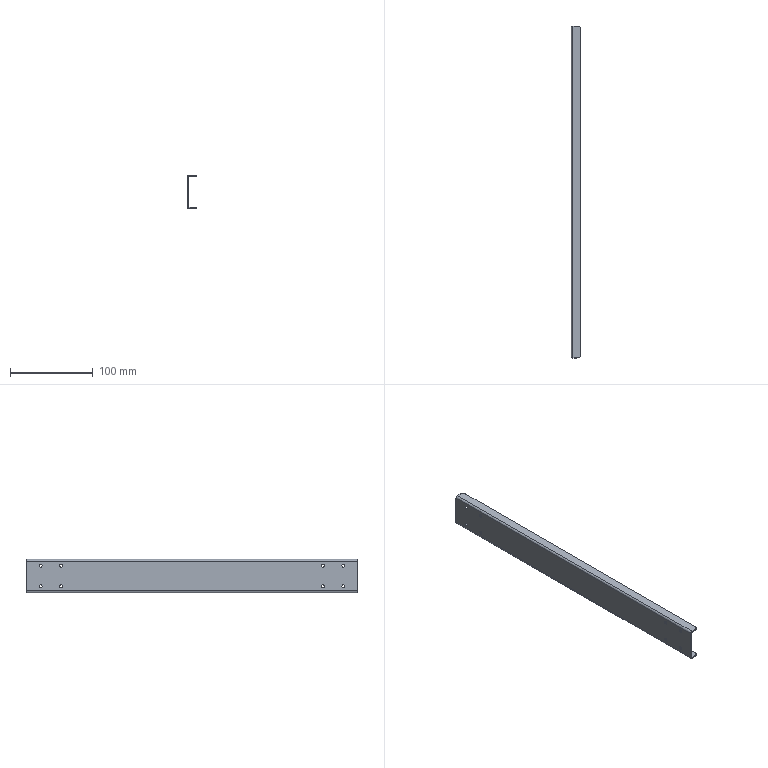Component | SolidWorks | 017-1 | 1 solid | 42 faces | volume 35550 mm3 | plane 18 | cone 16 | cylinder 8 | commonest cylinder face diameters 10 x4 4.473 x2 1.473 x2 | material SUS304